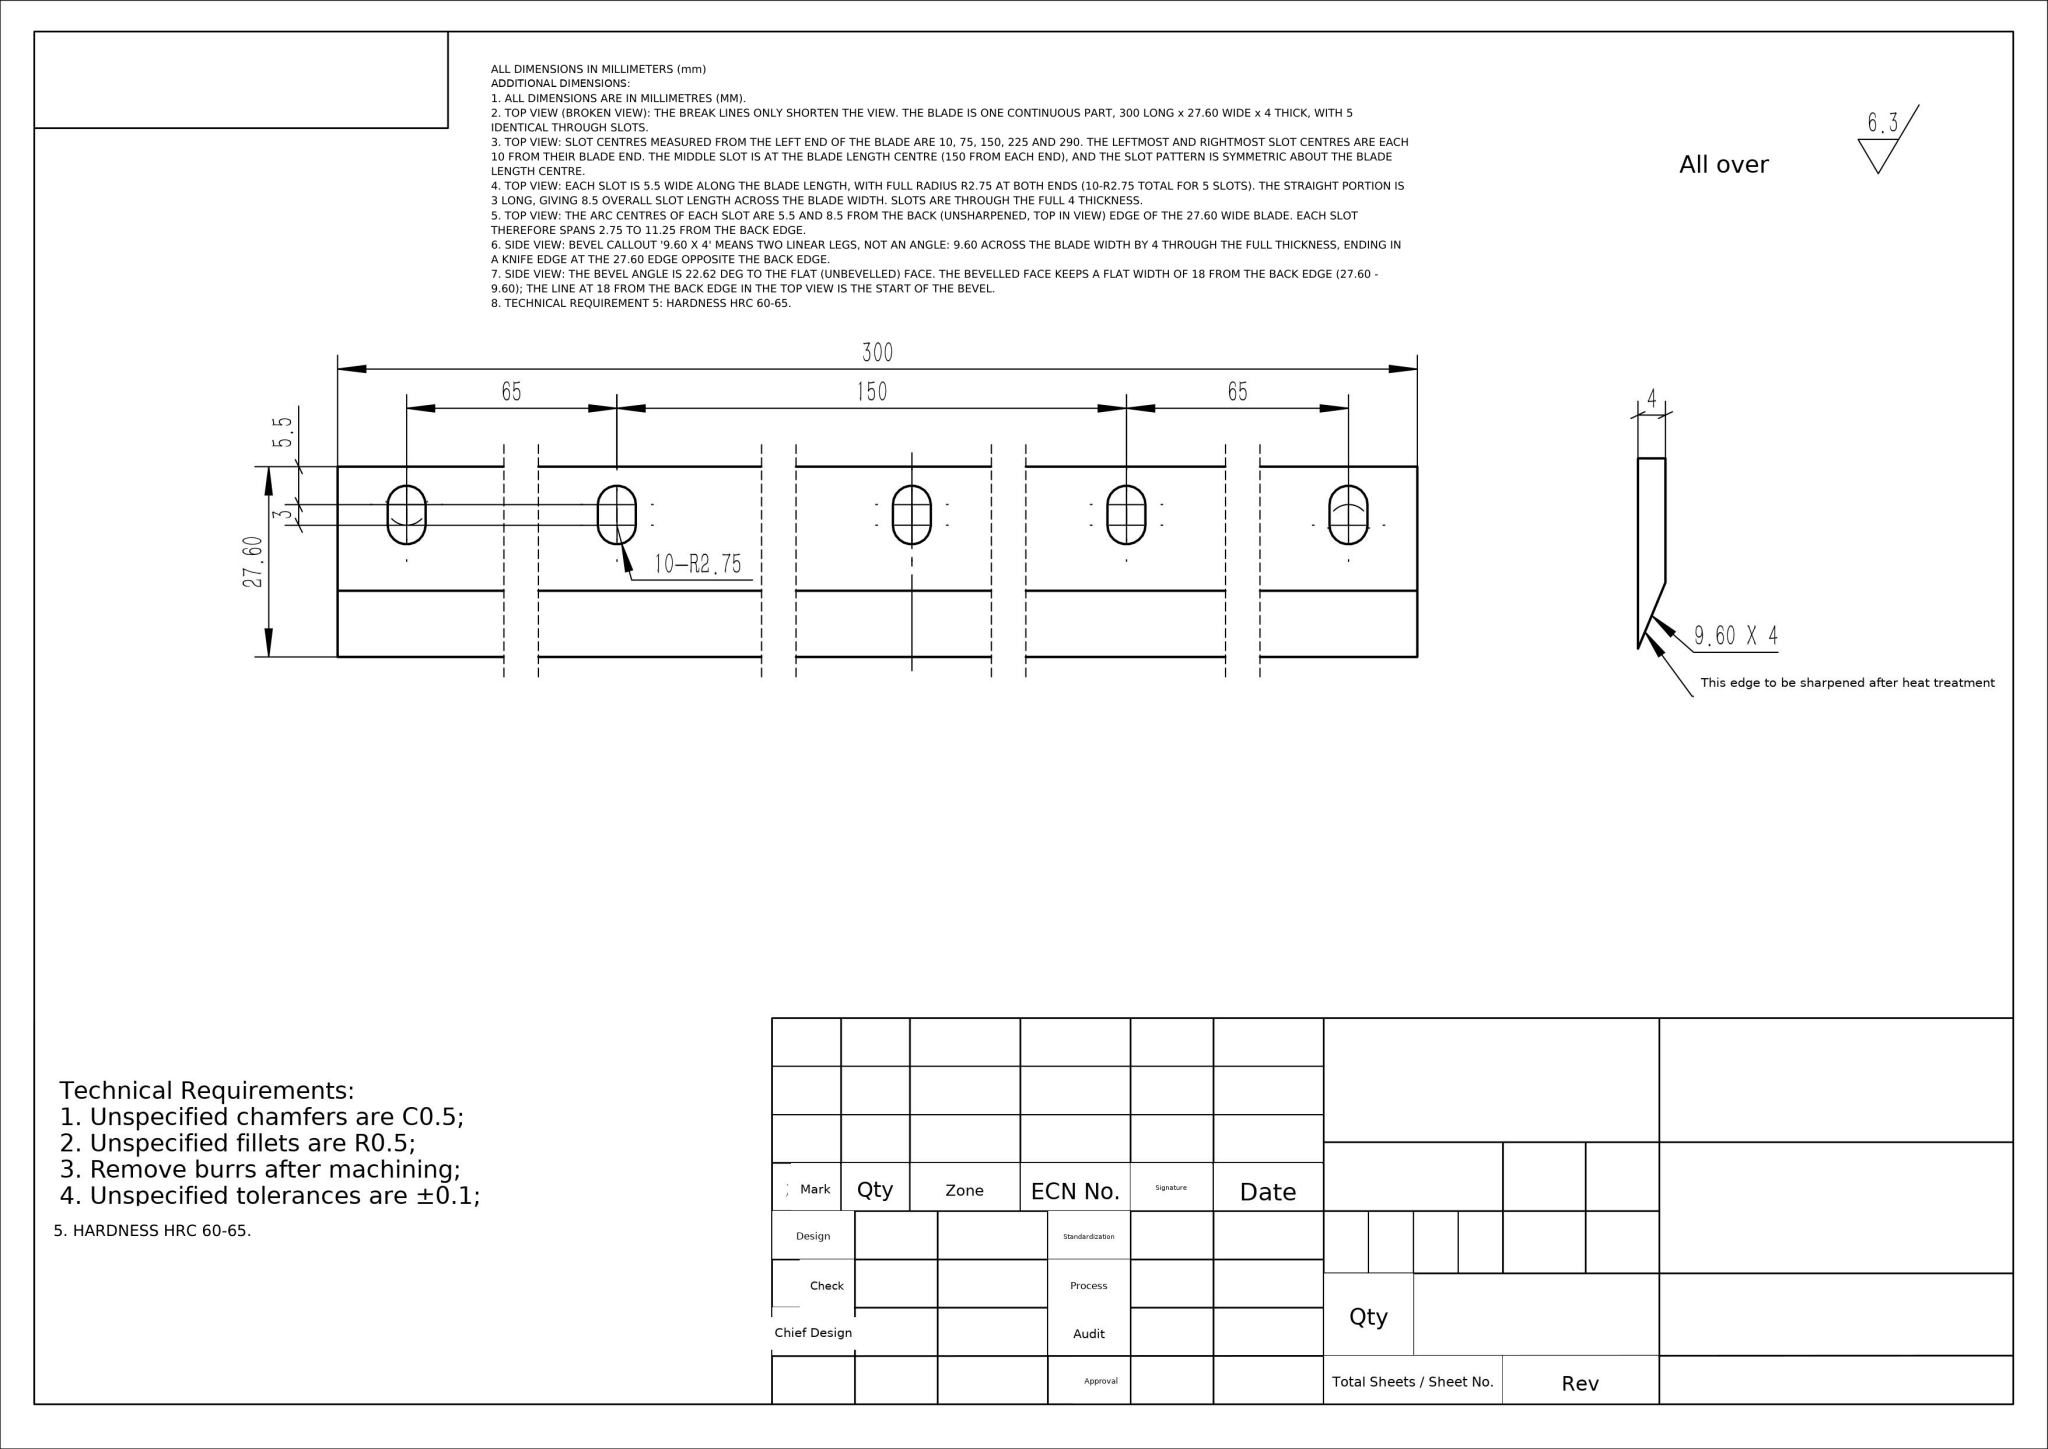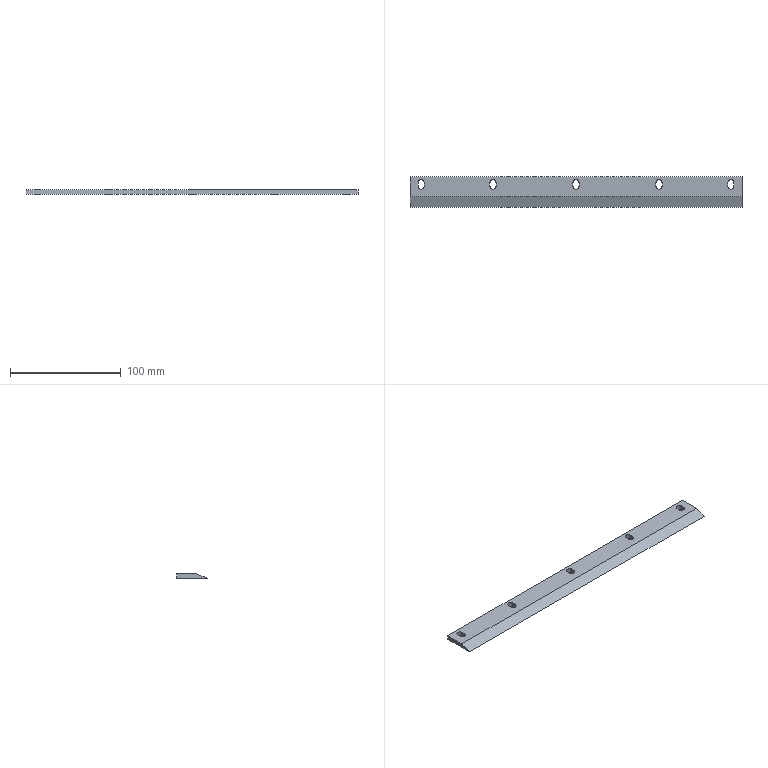Part | NX | mm | 479 | 1 solid | 26 faces | box 300 x 27.6 x 4 mm | volume 26555 mm3 | plane 16 | cylinder 10 | commonest cylinder face diameters 5.5 x10
STEP:
#1=COLOUR_RGB('',1.,1.,1.);
#2=FILL_AREA_STYLE_COLOUR('',#1);
#3=FILL_AREA_STYLE('',(#2));
#4=SURFACE_STYLE_FILL_AREA(#3);
#5=SURFACE_SIDE_STYLE('',(#4));
#6=SURFACE_STYLE_USAGE(.BOTH.,#5);
#7=PRESENTATION_STYLE_ASSIGNMENT((#6));
#8=CARTESIAN_POINT('',(-150.,0.,-2.));
#9=VERTEX_POINT('',#8);
#10=CARTESIAN_POINT('',(-150.,-27.6,-2.));
#11=VERTEX_POINT('',#10);
#12=CARTESIAN_POINT('',(-150.,0.,-2.));
#13=DIRECTION('',(0.,-1.,0.));
#14=VECTOR('',#13,1000.);
#15=LINE('',#12,#14);
#16=EDGE_CURVE('',#9,#11,#15,.T.);
#17=ORIENTED_EDGE('',*,*,#16,.T.);
#18=CARTESIAN_POINT('',(-150.,-18.,2.));
#19=VERTEX_POINT('',#18);
#20=CARTESIAN_POINT('',(-150.,-18.,2.));
#21=DIRECTION('',(0.,0.9231,0.3846));
#22=VECTOR('',#21,1000.);
#23=LINE('',#20,#22);
#24=EDGE_CURVE('',#11,#19,#23,.T.);
#25=ORIENTED_EDGE('',*,*,#24,.T.);
#26=CARTESIAN_POINT('',(-150.,0.,2.));
#27=VERTEX_POINT('',#26);
#28=CARTESIAN_POINT('',(-150.,0.,2.));
#29=DIRECTION('',(0.,-1.,0.));
#30=VECTOR('',#29,1000.);
#31=LINE('',#28,#30);
#32=EDGE_CURVE('',#27,#19,#31,.T.);
#33=ORIENTED_EDGE('',*,*,#32,.F.);
#34=CARTESIAN_POINT('',(-150.,0.,2.));
#35=DIRECTION('',(0.,0.,-1.));
#36=VECTOR('',#35,1000.);
#37=LINE('',#34,#36);
#38=EDGE_CURVE('',#27,#9,#37,.T.);
#39=ORIENTED_EDGE('',*,*,#38,.T.);
#40=EDGE_LOOP('',(#17,#25,#33,#39));
#41=FACE_OUTER_BOUND('',#40,.T.);
#42=CARTESIAN_POINT('',(-150.,0.,2.));
#43=DIRECTION('',(1.,0.,0.));
#44=DIRECTION('',(0.,0.,-1.));
#45=AXIS2_PLACEMENT_3D('',#42,#43,#44);
#46=PLANE('',#45);
#47=ADVANCED_FACE('',(#41),#46,.F.);
#48=CARTESIAN_POINT('',(150.,-18.,2.));
#49=VERTEX_POINT('',#48);
#50=CARTESIAN_POINT('',(150.,0.,2.));
#51=VERTEX_POINT('',#50);
#52=CARTESIAN_POINT('',(150.,-30.,2.));
#53=DIRECTION('',(0.,1.,0.));
#54=VECTOR('',#53,1000.);
#55=LINE('',#52,#54);
#56=EDGE_CURVE('',#49,#51,#55,.T.);
#57=ORIENTED_EDGE('',*,*,#56,.F.);
#58=CARTESIAN_POINT('',(150.,-27.6,-2.));
#59=VERTEX_POINT('',#58);
#60=CARTESIAN_POINT('',(150.,-18.,2.));
#61=DIRECTION('',(0.,-0.9231,-0.3846));
#62=VECTOR('',#61,1000.);
#63=LINE('',#60,#62);
#64=EDGE_CURVE('',#49,#59,#63,.T.);
#65=ORIENTED_EDGE('',*,*,#64,.T.);
#66=CARTESIAN_POINT('',(150.,0.,-2.));
#67=VERTEX_POINT('',#66);
#68=CARTESIAN_POINT('',(150.,-30.,-2.));
#69=DIRECTION('',(0.,1.,0.));
#70=VECTOR('',#69,1000.);
#71=LINE('',#68,#70);
#72=EDGE_CURVE('',#59,#67,#71,.T.);
#73=ORIENTED_EDGE('',*,*,#72,.T.);
#74=CARTESIAN_POINT('',(150.,0.,2.));
#75=DIRECTION('',(0.,0.,-1.));
#76=VECTOR('',#75,1000.);
#77=LINE('',#74,#76);
#78=EDGE_CURVE('',#51,#67,#77,.T.);
#79=ORIENTED_EDGE('',*,*,#78,.F.);
#80=EDGE_LOOP('',(#57,#65,#73,#79));
#81=FACE_OUTER_BOUND('',#80,.T.);
#82=CARTESIAN_POINT('',(150.,-30.,2.));
#83=DIRECTION('',(-1.,0.,0.));
#84=DIRECTION('',(0.,0.,1.));
#85=AXIS2_PLACEMENT_3D('',#82,#83,#84);
#86=PLANE('',#85);
#87=ADVANCED_FACE('',(#81),#86,.F.);
#88=CARTESIAN_POINT('',(-150.,0.,-2.));
#89=DIRECTION('',(-1.,0.,0.));
#90=VECTOR('',#89,1000.);
#91=LINE('',#88,#90);
#92=EDGE_CURVE('',#67,#9,#91,.T.);
#93=ORIENTED_EDGE('',*,*,#92,.T.);
#94=ORIENTED_EDGE('',*,*,#38,.F.);
#95=CARTESIAN_POINT('',(-150.,0.,2.));
#96=DIRECTION('',(-1.,0.,0.));
#97=VECTOR('',#96,1000.);
#98=LINE('',#95,#97);
#99=EDGE_CURVE('',#51,#27,#98,.T.);
#100=ORIENTED_EDGE('',*,*,#99,.F.);
#101=ORIENTED_EDGE('',*,*,#78,.T.);
#102=EDGE_LOOP('',(#93,#94,#100,#101));
#103=FACE_OUTER_BOUND('',#102,.T.);
#104=CARTESIAN_POINT('',(-150.,0.,2.));
#105=DIRECTION('',(0.,-1.,0.));
#106=DIRECTION('',(0.,0.,-1.));
#107=AXIS2_PLACEMENT_3D('',#104,#105,#106);
#108=PLANE('',#107);
#109=ADVANCED_FACE('',(#103),#108,.F.);
#110=CARTESIAN_POINT('',(142.75,-5.5,2.));
#111=VERTEX_POINT('',#110);
#112=CARTESIAN_POINT('',(137.25,-5.5,2.));
#113=VERTEX_POINT('',#112);
#114=CARTESIAN_POINT('',(140.,-5.5,2.));
#115=DIRECTION('',(0.,0.,1.));
#116=DIRECTION('',(-1.,0.,0.));
#117=AXIS2_PLACEMENT_3D('',#114,#115,#116);
#118=CIRCLE('',#117,2.75);
#119=EDGE_CURVE('',#111,#113,#118,.T.);
#120=ORIENTED_EDGE('',*,*,#119,.F.);
#121=CARTESIAN_POINT('',(142.75,-8.5,2.));
#122=VERTEX_POINT('',#121);
#123=CARTESIAN_POINT('',(142.75,-5.5,2.));
#124=DIRECTION('',(0.,1.,0.));
#125=VECTOR('',#124,1000.);
#126=LINE('',#123,#125);
#127=EDGE_CURVE('',#122,#111,#126,.T.);
#128=ORIENTED_EDGE('',*,*,#127,.F.);
#129=CARTESIAN_POINT('',(137.25,-8.5,2.));
#130=VERTEX_POINT('',#129);
#131=CARTESIAN_POINT('',(140.,-8.5,2.));
#132=DIRECTION('',(0.,0.,1.));
#133=DIRECTION('',(-1.,0.,0.));
#134=AXIS2_PLACEMENT_3D('',#131,#132,#133);
#135=CIRCLE('',#134,2.75);
#136=EDGE_CURVE('',#130,#122,#135,.T.);
#137=ORIENTED_EDGE('',*,*,#136,.F.);
#138=CARTESIAN_POINT('',(137.25,-5.5,2.));
#139=DIRECTION('',(0.,-1.,0.));
#140=VECTOR('',#139,1000.);
#141=LINE('',#138,#140);
#142=EDGE_CURVE('',#113,#130,#141,.T.);
#143=ORIENTED_EDGE('',*,*,#142,.F.);
#144=EDGE_LOOP('',(#120,#128,#137,#143));
#145=FACE_BOUND('',#144,.T.);
#146=CARTESIAN_POINT('',(-137.25,-5.5,2.));
#147=VERTEX_POINT('',#146);
#148=CARTESIAN_POINT('',(-142.75,-5.5,2.));
#149=VERTEX_POINT('',#148);
#150=CARTESIAN_POINT('',(-140.,-5.5,2.));
#151=DIRECTION('',(0.,0.,1.));
#152=DIRECTION('',(1.,0.,0.));
#153=AXIS2_PLACEMENT_3D('',#150,#151,#152);
#154=CIRCLE('',#153,2.75);
#155=EDGE_CURVE('',#147,#149,#154,.T.);
#156=ORIENTED_EDGE('',*,*,#155,.F.);
#157=CARTESIAN_POINT('',(-137.25,-8.5,2.));
#158=VERTEX_POINT('',#157);
#159=CARTESIAN_POINT('',(-137.25,-5.5,2.));
#160=DIRECTION('',(0.,1.,0.));
#161=VECTOR('',#160,1000.);
#162=LINE('',#159,#161);
#163=EDGE_CURVE('',#158,#147,#162,.T.);
#164=ORIENTED_EDGE('',*,*,#163,.F.);
#165=CARTESIAN_POINT('',(-142.75,-8.5,2.));
#166=VERTEX_POINT('',#165);
#167=CARTESIAN_POINT('',(-140.,-8.5,2.));
#168=DIRECTION('',(0.,0.,1.));
#169=DIRECTION('',(1.,0.,0.));
#170=AXIS2_PLACEMENT_3D('',#167,#168,#169);
#171=CIRCLE('',#170,2.75);
#172=EDGE_CURVE('',#166,#158,#171,.T.);
#173=ORIENTED_EDGE('',*,*,#172,.F.);
#174=CARTESIAN_POINT('',(-142.75,-5.5,2.));
#175=DIRECTION('',(0.,-1.,0.));
#176=VECTOR('',#175,1000.);
#177=LINE('',#174,#176);
#178=EDGE_CURVE('',#149,#166,#177,.T.);
#179=ORIENTED_EDGE('',*,*,#178,.F.);
#180=EDGE_LOOP('',(#156,#164,#173,#179));
#181=FACE_BOUND('',#180,.T.);
#182=CARTESIAN_POINT('',(2.75,-5.5,2.));
#183=VERTEX_POINT('',#182);
#184=CARTESIAN_POINT('',(-2.75,-5.5,2.));
#185=VERTEX_POINT('',#184);
#186=CARTESIAN_POINT('',(-0.,-5.5,2.));
#187=DIRECTION('',(0.,0.,1.));
#188=DIRECTION('',(1.,0.,0.));
#189=AXIS2_PLACEMENT_3D('',#186,#187,#188);
#190=CIRCLE('',#189,2.75);
#191=EDGE_CURVE('',#183,#185,#190,.T.);
#192=ORIENTED_EDGE('',*,*,#191,.F.);
#193=CARTESIAN_POINT('',(2.75,-8.5,2.));
#194=VERTEX_POINT('',#193);
#195=CARTESIAN_POINT('',(2.75,-5.5,2.));
#196=DIRECTION('',(-0.,1.,0.));
#197=VECTOR('',#196,1000.);
#198=LINE('',#195,#197);
#199=EDGE_CURVE('',#194,#183,#198,.T.);
#200=ORIENTED_EDGE('',*,*,#199,.F.);
#201=CARTESIAN_POINT('',(-2.75,-8.5,2.));
#202=VERTEX_POINT('',#201);
#203=CARTESIAN_POINT('',(0.,-8.5,2.));
#204=DIRECTION('',(0.,0.,1.));
#205=DIRECTION('',(1.,0.,0.));
#206=AXIS2_PLACEMENT_3D('',#203,#204,#205);
#207=CIRCLE('',#206,2.75);
#208=EDGE_CURVE('',#202,#194,#207,.T.);
#209=ORIENTED_EDGE('',*,*,#208,.F.);
#210=CARTESIAN_POINT('',(-2.75,-5.5,2.));
#211=DIRECTION('',(0.,-1.,0.));
#212=VECTOR('',#211,1000.);
#213=LINE('',#210,#212);
#214=EDGE_CURVE('',#185,#202,#213,.T.);
#215=ORIENTED_EDGE('',*,*,#214,.F.);
#216=EDGE_LOOP('',(#192,#200,#209,#215));
#217=FACE_BOUND('',#216,.T.);
#218=CARTESIAN_POINT('',(77.75,-5.5,2.));
#219=VERTEX_POINT('',#218);
#220=CARTESIAN_POINT('',(72.25,-5.5,2.));
#221=VERTEX_POINT('',#220);
#222=CARTESIAN_POINT('',(75.,-5.5,2.));
#223=DIRECTION('',(0.,0.,1.));
#224=DIRECTION('',(-1.,0.,0.));
#225=AXIS2_PLACEMENT_3D('',#222,#223,#224);
#226=CIRCLE('',#225,2.75);
#227=EDGE_CURVE('',#219,#221,#226,.T.);
#228=ORIENTED_EDGE('',*,*,#227,.F.);
#229=CARTESIAN_POINT('',(77.75,-8.5,2.));
#230=VERTEX_POINT('',#229);
#231=CARTESIAN_POINT('',(77.75,-5.5,2.));
#232=DIRECTION('',(0.,1.,0.));
#233=VECTOR('',#232,1000.);
#234=LINE('',#231,#233);
#235=EDGE_CURVE('',#230,#219,#234,.T.);
#236=ORIENTED_EDGE('',*,*,#235,.F.);
#237=CARTESIAN_POINT('',(72.25,-8.5,2.));
#238=VERTEX_POINT('',#237);
#239=CARTESIAN_POINT('',(75.,-8.5,2.));
#240=DIRECTION('',(0.,0.,1.));
#241=DIRECTION('',(-1.,0.,0.));
#242=AXIS2_PLACEMENT_3D('',#239,#240,#241);
#243=CIRCLE('',#242,2.75);
#244=EDGE_CURVE('',#238,#230,#243,.T.);
#245=ORIENTED_EDGE('',*,*,#244,.F.);
#246=CARTESIAN_POINT('',(72.25,-5.5,2.));
#247=DIRECTION('',(0.,-1.,0.));
#248=VECTOR('',#247,1000.);
#249=LINE('',#246,#248);
#250=EDGE_CURVE('',#221,#238,#249,.T.);
#251=ORIENTED_EDGE('',*,*,#250,.F.);
#252=EDGE_LOOP('',(#228,#236,#245,#251));
#253=FACE_BOUND('',#252,.T.);
#254=CARTESIAN_POINT('',(-72.25,-5.5,2.));
#255=VERTEX_POINT('',#254);
#256=CARTESIAN_POINT('',(-77.75,-5.5,2.));
#257=VERTEX_POINT('',#256);
#258=CARTESIAN_POINT('',(-75.,-5.5,2.));
#259=DIRECTION('',(0.,0.,1.));
#260=DIRECTION('',(1.,0.,0.));
#261=AXIS2_PLACEMENT_3D('',#258,#259,#260);
#262=CIRCLE('',#261,2.75);
#263=EDGE_CURVE('',#255,#257,#262,.T.);
#264=ORIENTED_EDGE('',*,*,#263,.F.);
#265=CARTESIAN_POINT('',(-72.25,-8.5,2.));
#266=VERTEX_POINT('',#265);
#267=CARTESIAN_POINT('',(-72.25,-5.5,2.));
#268=DIRECTION('',(0.,1.,0.));
#269=VECTOR('',#268,1000.);
#270=LINE('',#267,#269);
#271=EDGE_CURVE('',#266,#255,#270,.T.);
#272=ORIENTED_EDGE('',*,*,#271,.F.);
#273=CARTESIAN_POINT('',(-77.75,-8.5,2.));
#274=VERTEX_POINT('',#273);
#275=CARTESIAN_POINT('',(-75.,-8.5,2.));
#276=DIRECTION('',(0.,0.,1.));
#277=DIRECTION('',(1.,0.,0.));
#278=AXIS2_PLACEMENT_3D('',#275,#276,#277);
#279=CIRCLE('',#278,2.75);
#280=EDGE_CURVE('',#274,#266,#279,.T.);
#281=ORIENTED_EDGE('',*,*,#280,.F.);
#282=CARTESIAN_POINT('',(-77.75,-5.5,2.));
#283=DIRECTION('',(0.,-1.,0.));
#284=VECTOR('',#283,1000.);
#285=LINE('',#282,#284);
#286=EDGE_CURVE('',#257,#274,#285,.T.);
#287=ORIENTED_EDGE('',*,*,#286,.F.);
#288=EDGE_LOOP('',(#264,#272,#281,#287));
#289=FACE_BOUND('',#288,.T.);
#290=ORIENTED_EDGE('',*,*,#32,.T.);
#291=CARTESIAN_POINT('',(150.,-18.,2.));
#292=DIRECTION('',(1.,0.,0.));
#293=VECTOR('',#292,1000.);
#294=LINE('',#291,#293);
#295=EDGE_CURVE('',#19,#49,#294,.T.);
#296=ORIENTED_EDGE('',*,*,#295,.T.);
#297=ORIENTED_EDGE('',*,*,#56,.T.);
#298=ORIENTED_EDGE('',*,*,#99,.T.);
#299=EDGE_LOOP('',(#290,#296,#297,#298));
#300=FACE_OUTER_BOUND('',#299,.T.);
#301=CARTESIAN_POINT('',(0.,0.,2.));
#302=DIRECTION('',(0.,0.,1.));
#303=DIRECTION('',(1.,0.,0.));
#304=AXIS2_PLACEMENT_3D('',#301,#302,#303);
#305=PLANE('',#304);
#306=ADVANCED_FACE('',(#145,#181,#217,#253,#289,#300),#305,.T.);
#307=CARTESIAN_POINT('',(142.75,-8.5,-2.));
#308=VERTEX_POINT('',#307);
#309=CARTESIAN_POINT('',(142.75,-5.5,-2.));
#310=VERTEX_POINT('',#309);
#311=CARTESIAN_POINT('',(142.75,-5.5,-2.));
#312=DIRECTION('',(0.,1.,0.));
#313=VECTOR('',#312,1000.);
#314=LINE('',#311,#313);
#315=EDGE_CURVE('',#308,#310,#314,.T.);
#316=ORIENTED_EDGE('',*,*,#315,.T.);
#317=CARTESIAN_POINT('',(137.25,-5.5,-2.));
#318=VERTEX_POINT('',#317);
#319=CARTESIAN_POINT('',(140.,-5.5,-2.));
#320=DIRECTION('',(0.,0.,1.));
#321=DIRECTION('',(-1.,0.,0.));
#322=AXIS2_PLACEMENT_3D('',#319,#320,#321);
#323=CIRCLE('',#322,2.75);
#324=EDGE_CURVE('',#310,#318,#323,.T.);
#325=ORIENTED_EDGE('',*,*,#324,.T.);
#326=CARTESIAN_POINT('',(137.25,-8.5,-2.));
#327=VERTEX_POINT('',#326);
#328=CARTESIAN_POINT('',(137.25,-5.5,-2.));
#329=DIRECTION('',(0.,-1.,0.));
#330=VECTOR('',#329,1000.);
#331=LINE('',#328,#330);
#332=EDGE_CURVE('',#318,#327,#331,.T.);
#333=ORIENTED_EDGE('',*,*,#332,.T.);
#334=CARTESIAN_POINT('',(140.,-8.5,-2.));
#335=DIRECTION('',(0.,0.,1.));
#336=DIRECTION('',(-1.,0.,0.));
#337=AXIS2_PLACEMENT_3D('',#334,#335,#336);
#338=CIRCLE('',#337,2.75);
#339=EDGE_CURVE('',#327,#308,#338,.T.);
#340=ORIENTED_EDGE('',*,*,#339,.T.);
#341=EDGE_LOOP('',(#316,#325,#333,#340));
#342=FACE_BOUND('',#341,.T.);
#343=CARTESIAN_POINT('',(-137.25,-8.5,-2.));
#344=VERTEX_POINT('',#343);
#345=CARTESIAN_POINT('',(-137.25,-5.5,-2.));
#346=VERTEX_POINT('',#345);
#347=CARTESIAN_POINT('',(-137.25,-5.5,-2.));
#348=DIRECTION('',(0.,1.,0.));
#349=VECTOR('',#348,1000.);
#350=LINE('',#347,#349);
#351=EDGE_CURVE('',#344,#346,#350,.T.);
#352=ORIENTED_EDGE('',*,*,#351,.T.);
#353=CARTESIAN_POINT('',(-142.75,-5.5,-2.));
#354=VERTEX_POINT('',#353);
#355=CARTESIAN_POINT('',(-140.,-5.5,-2.));
#356=DIRECTION('',(0.,0.,1.));
#357=DIRECTION('',(1.,0.,0.));
#358=AXIS2_PLACEMENT_3D('',#355,#356,#357);
#359=CIRCLE('',#358,2.75);
#360=EDGE_CURVE('',#346,#354,#359,.T.);
#361=ORIENTED_EDGE('',*,*,#360,.T.);
#362=CARTESIAN_POINT('',(-142.75,-8.5,-2.));
#363=VERTEX_POINT('',#362);
#364=CARTESIAN_POINT('',(-142.75,-5.5,-2.));
#365=DIRECTION('',(0.,-1.,0.));
#366=VECTOR('',#365,1000.);
#367=LINE('',#364,#366);
#368=EDGE_CURVE('',#354,#363,#367,.T.);
#369=ORIENTED_EDGE('',*,*,#368,.T.);
#370=CARTESIAN_POINT('',(-140.,-8.5,-2.));
#371=DIRECTION('',(0.,0.,1.));
#372=DIRECTION('',(1.,0.,0.));
#373=AXIS2_PLACEMENT_3D('',#370,#371,#372);
#374=CIRCLE('',#373,2.75);
#375=EDGE_CURVE('',#363,#344,#374,.T.);
#376=ORIENTED_EDGE('',*,*,#375,.T.);
#377=EDGE_LOOP('',(#352,#361,#369,#376));
#378=FACE_BOUND('',#377,.T.);
#379=CARTESIAN_POINT('',(2.75,-8.5,-2.));
#380=VERTEX_POINT('',#379);
#381=CARTESIAN_POINT('',(2.75,-5.5,-2.));
#382=VERTEX_POINT('',#381);
#383=CARTESIAN_POINT('',(2.75,-5.5,-2.));
#384=DIRECTION('',(-0.,1.,0.));
#385=VECTOR('',#384,1000.);
#386=LINE('',#383,#385);
#387=EDGE_CURVE('',#380,#382,#386,.T.);
#388=ORIENTED_EDGE('',*,*,#387,.T.);
#389=CARTESIAN_POINT('',(-2.75,-5.5,-2.));
#390=VERTEX_POINT('',#389);
#391=CARTESIAN_POINT('',(-0.,-5.5,-2.));
#392=DIRECTION('',(0.,0.,1.));
#393=DIRECTION('',(1.,0.,0.));
#394=AXIS2_PLACEMENT_3D('',#391,#392,#393);
#395=CIRCLE('',#394,2.75);
#396=EDGE_CURVE('',#382,#390,#395,.T.);
#397=ORIENTED_EDGE('',*,*,#396,.T.);
#398=CARTESIAN_POINT('',(-2.75,-8.5,-2.));
#399=VERTEX_POINT('',#398);
#400=CARTESIAN_POINT('',(-2.75,-5.5,-2.));
#401=DIRECTION('',(0.,-1.,0.));
#402=VECTOR('',#401,1000.);
#403=LINE('',#400,#402);
#404=EDGE_CURVE('',#390,#399,#403,.T.);
#405=ORIENTED_EDGE('',*,*,#404,.T.);
#406=CARTESIAN_POINT('',(0.,-8.5,-2.));
#407=DIRECTION('',(0.,0.,1.));
#408=DIRECTION('',(1.,0.,0.));
#409=AXIS2_PLACEMENT_3D('',#406,#407,#408);
#410=CIRCLE('',#409,2.75);
#411=EDGE_CURVE('',#399,#380,#410,.T.);
#412=ORIENTED_EDGE('',*,*,#411,.T.);
#413=EDGE_LOOP('',(#388,#397,#405,#412));
#414=FACE_BOUND('',#413,.T.);
#415=CARTESIAN_POINT('',(77.75,-8.5,-2.));
#416=VERTEX_POINT('',#415);
#417=CARTESIAN_POINT('',(77.75,-5.5,-2.));
#418=VERTEX_POINT('',#417);
#419=CARTESIAN_POINT('',(77.75,-5.5,-2.));
#420=DIRECTION('',(0.,1.,0.));
#421=VECTOR('',#420,1000.);
#422=LINE('',#419,#421);
#423=EDGE_CURVE('',#416,#418,#422,.T.);
#424=ORIENTED_EDGE('',*,*,#423,.T.);
#425=CARTESIAN_POINT('',(72.25,-5.5,-2.));
#426=VERTEX_POINT('',#425);
#427=CARTESIAN_POINT('',(75.,-5.5,-2.));
#428=DIRECTION('',(0.,0.,1.));
#429=DIRECTION('',(-1.,0.,0.));
#430=AXIS2_PLACEMENT_3D('',#427,#428,#429);
#431=CIRCLE('',#430,2.75);
#432=EDGE_CURVE('',#418,#426,#431,.T.);
#433=ORIENTED_EDGE('',*,*,#432,.T.);
#434=CARTESIAN_POINT('',(72.25,-8.5,-2.));
#435=VERTEX_POINT('',#434);
#436=CARTESIAN_POINT('',(72.25,-5.5,-2.));
#437=DIRECTION('',(0.,-1.,0.));
#438=VECTOR('',#437,1000.);
#439=LINE('',#436,#438);
#440=EDGE_CURVE('',#426,#435,#439,.T.);
#441=ORIENTED_EDGE('',*,*,#440,.T.);
#442=CARTESIAN_POINT('',(75.,-8.5,-2.));
#443=DIRECTION('',(0.,0.,1.));
#444=DIRECTION('',(-1.,0.,0.));
#445=AXIS2_PLACEMENT_3D('',#442,#443,#444);
#446=CIRCLE('',#445,2.75);
#447=EDGE_CURVE('',#435,#416,#446,.T.);
#448=ORIENTED_EDGE('',*,*,#447,.T.);
#449=EDGE_LOOP('',(#424,#433,#441,#448));
#450=FACE_BOUND('',#449,.T.);
#451=CARTESIAN_POINT('',(-72.25,-8.5,-2.));
#452=VERTEX_POINT('',#451);
#453=CARTESIAN_POINT('',(-72.25,-5.5,-2.));
#454=VERTEX_POINT('',#453);
#455=CARTESIAN_POINT('',(-72.25,-5.5,-2.));
#456=DIRECTION('',(0.,1.,0.));
#457=VECTOR('',#456,1000.);
#458=LINE('',#455,#457);
#459=EDGE_CURVE('',#452,#454,#458,.T.);
#460=ORIENTED_EDGE('',*,*,#459,.T.);
#461=CARTESIAN_POINT('',(-77.75,-5.5,-2.));
#462=VERTEX_POINT('',#461);
#463=CARTESIAN_POINT('',(-75.,-5.5,-2.));
#464=DIRECTION('',(0.,0.,1.));
#465=DIRECTION('',(1.,0.,0.));
#466=AXIS2_PLACEMENT_3D('',#463,#464,#465);
#467=CIRCLE('',#466,2.75);
#468=EDGE_CURVE('',#454,#462,#467,.T.);
#469=ORIENTED_EDGE('',*,*,#468,.T.);
#470=CARTESIAN_POINT('',(-77.75,-8.5,-2.));
#471=VERTEX_POINT('',#470);
#472=CARTESIAN_POINT('',(-77.75,-5.5,-2.));
#473=DIRECTION('',(0.,-1.,0.));
#474=VECTOR('',#473,1000.);
#475=LINE('',#472,#474);
#476=EDGE_CURVE('',#462,#471,#475,.T.);
#477=ORIENTED_EDGE('',*,*,#476,.T.);
#478=CARTESIAN_POINT('',(-75.,-8.5,-2.));
#479=DIRECTION('',(0.,0.,1.));
#480=DIRECTION('',(1.,0.,0.));
#481=AXIS2_PLACEMENT_3D('',#478,#479,#480);
#482=CIRCLE('',#481,2.75);
#483=EDGE_CURVE('',#471,#452,#482,.T.);
#484=ORIENTED_EDGE('',*,*,#483,.T.);
#485=EDGE_LOOP('',(#460,#469,#477,#484));
#486=FACE_BOUND('',#485,.T.);
#487=ORIENTED_EDGE('',*,*,#72,.F.);
#488=CARTESIAN_POINT('',(0.,-27.6,-2.));
#489=DIRECTION('',(-1.,0.,0.));
#490=VECTOR('',#489,1000.);
#491=LINE('',#488,#490);
#492=EDGE_CURVE('',#59,#11,#491,.T.);
#493=ORIENTED_EDGE('',*,*,#492,.T.);
#494=ORIENTED_EDGE('',*,*,#16,.F.);
#495=ORIENTED_EDGE('',*,*,#92,.F.);
#496=EDGE_LOOP('',(#487,#493,#494,#495));
#497=FACE_OUTER_BOUND('',#496,.T.);
#498=CARTESIAN_POINT('',(0.,0.,-2.));
#499=DIRECTION('',(0.,0.,1.));
#500=DIRECTION('',(1.,0.,0.));
#501=AXIS2_PLACEMENT_3D('',#498,#499,#500);
#502=PLANE('',#501);
#503=ADVANCED_FACE('',(#342,#378,#414,#450,#486,#497),#502,.F.);
#504=ORIENTED_EDGE('',*,*,#24,.F.);
#505=ORIENTED_EDGE('',*,*,#492,.F.);
#506=ORIENTED_EDGE('',*,*,#64,.F.);
#507=ORIENTED_EDGE('',*,*,#295,.F.);
#508=EDGE_LOOP('',(#504,#505,#506,#507));
#509=FACE_OUTER_BOUND('',#508,.T.);
#510=CARTESIAN_POINT('',(0.,-18.,2.));
#511=DIRECTION('',(0.,-0.3846,0.9231));
#512=DIRECTION('',(-1.,0.,0.));
#513=AXIS2_PLACEMENT_3D('',#510,#511,#512);
#514=PLANE('',#513);
#515=ADVANCED_FACE('',(#509),#514,.T.);
#516=ORIENTED_EDGE('',*,*,#263,.T.);
#517=CARTESIAN_POINT('',(-77.75,-5.5,-2.));
#518=DIRECTION('',(0.,0.,1.));
#519=VECTOR('',#518,1000.);
#520=LINE('',#517,#519);
#521=EDGE_CURVE('',#462,#257,#520,.T.);
#522=ORIENTED_EDGE('',*,*,#521,.F.);
#523=ORIENTED_EDGE('',*,*,#468,.F.);
#524=CARTESIAN_POINT('',(-72.25,-5.5,-2.));
#525=DIRECTION('',(0.,0.,1.));
#526=VECTOR('',#525,1000.);
#527=LINE('',#524,#526);
#528=EDGE_CURVE('',#454,#255,#527,.T.);
#529=ORIENTED_EDGE('',*,*,#528,.T.);
#530=EDGE_LOOP('',(#516,#522,#523,#529));
#531=FACE_OUTER_BOUND('',#530,.T.);
#532=CARTESIAN_POINT('',(-75.,-5.5,-2.));
#533=DIRECTION('',(0.,0.,1.));
#534=DIRECTION('',(1.,0.,0.));
#535=AXIS2_PLACEMENT_3D('',#532,#533,#534);
#536=CYLINDRICAL_SURFACE('',#535,2.75);
#537=ADVANCED_FACE('',(#531),#536,.F.);
#538=ORIENTED_EDGE('',*,*,#271,.T.);
#539=ORIENTED_EDGE('',*,*,#528,.F.);
#540=ORIENTED_EDGE('',*,*,#459,.F.);
#541=CARTESIAN_POINT('',(-72.25,-8.5,-2.));
#542=DIRECTION('',(0.,0.,1.));
#543=VECTOR('',#542,1000.);
#544=LINE('',#541,#543);
#545=EDGE_CURVE('',#452,#266,#544,.T.);
#546=ORIENTED_EDGE('',*,*,#545,.T.);
#547=EDGE_LOOP('',(#538,#539,#540,#546));
#548=FACE_OUTER_BOUND('',#547,.T.);
#549=CARTESIAN_POINT('',(-72.25,-5.5,-2.));
#550=DIRECTION('',(1.,0.,0.));
#551=DIRECTION('',(0.,0.,-1.));
#552=AXIS2_PLACEMENT_3D('',#549,#550,#551);
#553=PLANE('',#552);
#554=ADVANCED_FACE('',(#548),#553,.F.);
#555=ORIENTED_EDGE('',*,*,#280,.T.);
#556=ORIENTED_EDGE('',*,*,#545,.F.);
#557=ORIENTED_EDGE('',*,*,#483,.F.);
#558=CARTESIAN_POINT('',(-77.75,-8.5,-2.));
#559=DIRECTION('',(0.,0.,1.));
#560=VECTOR('',#559,1000.);
#561=LINE('',#558,#560);
#562=EDGE_CURVE('',#471,#274,#561,.T.);
#563=ORIENTED_EDGE('',*,*,#562,.T.);
#564=EDGE_LOOP('',(#555,#556,#557,#563));
#565=FACE_OUTER_BOUND('',#564,.T.);
#566=CARTESIAN_POINT('',(-75.,-8.5,-2.));
#567=DIRECTION('',(0.,0.,1.));
#568=DIRECTION('',(1.,0.,0.));
#569=AXIS2_PLACEMENT_3D('',#566,#567,#568);
#570=CYLINDRICAL_SURFACE('',#569,2.75);
#571=ADVANCED_FACE('',(#565),#570,.F.);
#572=ORIENTED_EDGE('',*,*,#286,.T.);
#573=ORIENTED_EDGE('',*,*,#562,.F.);
#574=ORIENTED_EDGE('',*,*,#476,.F.);
#575=ORIENTED_EDGE('',*,*,#521,.T.);
#576=EDGE_LOOP('',(#572,#573,#574,#575));
#577=FACE_OUTER_BOUND('',#576,.T.);
#578=CARTESIAN_POINT('',(-77.75,-5.5,-2.));
#579=DIRECTION('',(-1.,0.,0.));
#580=DIRECTION('',(0.,0.,1.));
#581=AXIS2_PLACEMENT_3D('',#578,#579,#580);
#582=PLANE('',#581);
#583=ADVANCED_FACE('',(#577),#582,.F.);
#584=ORIENTED_EDGE('',*,*,#227,.T.);
#585=CARTESIAN_POINT('',(72.25,-5.5,-2.));
#586=DIRECTION('',(0.,0.,1.));
#587=VECTOR('',#586,1000.);
#588=LINE('',#585,#587);
#589=EDGE_CURVE('',#426,#221,#588,.T.);
#590=ORIENTED_EDGE('',*,*,#589,.F.);
#591=ORIENTED_EDGE('',*,*,#432,.F.);
#592=CARTESIAN_POINT('',(77.75,-5.5,-2.));
#593=DIRECTION('',(0.,0.,1.));
#594=VECTOR('',#593,1000.);
#595=LINE('',#592,#594);
#596=EDGE_CURVE('',#418,#219,#595,.T.);
#597=ORIENTED_EDGE('',*,*,#596,.T.);
#598=EDGE_LOOP('',(#584,#590,#591,#597));
#599=FACE_OUTER_BOUND('',#598,.T.);
#600=CARTESIAN_POINT('',(75.,-5.5,-2.));
#601=DIRECTION('',(0.,0.,1.));
#602=DIRECTION('',(1.,0.,0.));
#603=AXIS2_PLACEMENT_3D('',#600,#601,#602);
#604=CYLINDRICAL_SURFACE('',#603,2.75);
#605=ADVANCED_FACE('',(#599),#604,.F.);
#606=ORIENTED_EDGE('',*,*,#235,.T.);
#607=ORIENTED_EDGE('',*,*,#596,.F.);
#608=ORIENTED_EDGE('',*,*,#423,.F.);
#609=CARTESIAN_POINT('',(77.75,-8.5,-2.));
#610=DIRECTION('',(0.,0.,1.));
#611=VECTOR('',#610,1000.);
#612=LINE('',#609,#611);
#613=EDGE_CURVE('',#416,#230,#612,.T.);
#614=ORIENTED_EDGE('',*,*,#613,.T.);
#615=EDGE_LOOP('',(#606,#607,#608,#614));
#616=FACE_OUTER_BOUND('',#615,.T.);
#617=CARTESIAN_POINT('',(77.75,-5.5,-2.));
#618=DIRECTION('',(1.,0.,0.));
#619=DIRECTION('',(0.,0.,-1.));
#620=AXIS2_PLACEMENT_3D('',#617,#618,#619);
#621=PLANE('',#620);
#622=ADVANCED_FACE('',(#616),#621,.F.);
#623=ORIENTED_EDGE('',*,*,#244,.T.);
#624=ORIENTED_EDGE('',*,*,#613,.F.);
#625=ORIENTED_EDGE('',*,*,#447,.F.);
#626=CARTESIAN_POINT('',(72.25,-8.5,-2.));
#627=DIRECTION('',(0.,0.,1.));
#628=VECTOR('',#627,1000.);
#629=LINE('',#626,#628);
#630=EDGE_CURVE('',#435,#238,#629,.T.);
#631=ORIENTED_EDGE('',*,*,#630,.T.);
#632=EDGE_LOOP('',(#623,#624,#625,#631));
#633=FACE_OUTER_BOUND('',#632,.T.);
#634=CARTESIAN_POINT('',(75.,-8.5,-2.));
#635=DIRECTION('',(0.,0.,1.));
#636=DIRECTION('',(1.,0.,0.));
#637=AXIS2_PLACEMENT_3D('',#634,#635,#636);
#638=CYLINDRICAL_SURFACE('',#637,2.75);
#639=ADVANCED_FACE('',(#633),#638,.F.);
#640=ORIENTED_EDGE('',*,*,#250,.T.);
#641=ORIENTED_EDGE('',*,*,#630,.F.);
#642=ORIENTED_EDGE('',*,*,#440,.F.);
#643=ORIENTED_EDGE('',*,*,#589,.T.);
#644=EDGE_LOOP('',(#640,#641,#642,#643));
#645=FACE_OUTER_BOUND('',#644,.T.);
#646=CARTESIAN_POINT('',(72.25,-5.5,-2.));
#647=DIRECTION('',(-1.,0.,0.));
#648=DIRECTION('',(0.,0.,1.));
#649=AXIS2_PLACEMENT_3D('',#646,#647,#648);
#650=PLANE('',#649);
#651=ADVANCED_FACE('',(#645),#650,.F.);
#652=ORIENTED_EDGE('',*,*,#191,.T.);
#653=CARTESIAN_POINT('',(-2.75,-5.5,-2.));
#654=DIRECTION('',(0.,0.,1.));
#655=VECTOR('',#654,1000.);
#656=LINE('',#653,#655);
#657=EDGE_CURVE('',#390,#185,#656,.T.);
#658=ORIENTED_EDGE('',*,*,#657,.F.);
#659=ORIENTED_EDGE('',*,*,#396,.F.);
#660=CARTESIAN_POINT('',(2.75,-5.5,-2.));
#661=DIRECTION('',(0.,0.,1.));
#662=VECTOR('',#661,1000.);
#663=LINE('',#660,#662);
#664=EDGE_CURVE('',#382,#183,#663,.T.);
#665=ORIENTED_EDGE('',*,*,#664,.T.);
#666=EDGE_LOOP('',(#652,#658,#659,#665));
#667=FACE_OUTER_BOUND('',#666,.T.);
#668=CARTESIAN_POINT('',(-0.,-5.5,-2.));
#669=DIRECTION('',(0.,0.,1.));
#670=DIRECTION('',(1.,0.,0.));
#671=AXIS2_PLACEMENT_3D('',#668,#669,#670);
#672=CYLINDRICAL_SURFACE('',#671,2.75);
#673=ADVANCED_FACE('',(#667),#672,.F.);
#674=ORIENTED_EDGE('',*,*,#199,.T.);
#675=ORIENTED_EDGE('',*,*,#664,.F.);
#676=ORIENTED_EDGE('',*,*,#387,.F.);
#677=CARTESIAN_POINT('',(2.75,-8.5,-2.));
#678=DIRECTION('',(0.,0.,1.));
#679=VECTOR('',#678,1000.);
#680=LINE('',#677,#679);
#681=EDGE_CURVE('',#380,#194,#680,.T.);
#682=ORIENTED_EDGE('',*,*,#681,.T.);
#683=EDGE_LOOP('',(#674,#675,#676,#682));
#684=FACE_OUTER_BOUND('',#683,.T.);
#685=CARTESIAN_POINT('',(2.75,-5.5,-2.));
#686=DIRECTION('',(1.,0.,0.));
#687=DIRECTION('',(-0.,1.,0.));
#688=AXIS2_PLACEMENT_3D('',#685,#686,#687);
#689=PLANE('',#688);
#690=ADVANCED_FACE('',(#684),#689,.F.);
#691=ORIENTED_EDGE('',*,*,#208,.T.);
#692=ORIENTED_EDGE('',*,*,#681,.F.);
#693=ORIENTED_EDGE('',*,*,#411,.F.);
#694=CARTESIAN_POINT('',(-2.75,-8.5,-2.));
#695=DIRECTION('',(0.,0.,1.));
#696=VECTOR('',#695,1000.);
#697=LINE('',#694,#696);
#698=EDGE_CURVE('',#399,#202,#697,.T.);
#699=ORIENTED_EDGE('',*,*,#698,.T.);
#700=EDGE_LOOP('',(#691,#692,#693,#699));
#701=FACE_OUTER_BOUND('',#700,.T.);
#702=CARTESIAN_POINT('',(0.,-8.5,-2.));
#703=DIRECTION('',(0.,0.,1.));
#704=DIRECTION('',(1.,0.,0.));
#705=AXIS2_PLACEMENT_3D('',#702,#703,#704);
#706=CYLINDRICAL_SURFACE('',#705,2.75);
#707=ADVANCED_FACE('',(#701),#706,.F.);
#708=ORIENTED_EDGE('',*,*,#214,.T.);
#709=ORIENTED_EDGE('',*,*,#698,.F.);
#710=ORIENTED_EDGE('',*,*,#404,.F.);
#711=ORIENTED_EDGE('',*,*,#657,.T.);
#712=EDGE_LOOP('',(#708,#709,#710,#711));
#713=FACE_OUTER_BOUND('',#712,.T.);
#714=CARTESIAN_POINT('',(-2.75,-5.5,-2.));
#715=DIRECTION('',(-1.,-0.,0.));
#716=DIRECTION('',(0.,-1.,0.));
#717=AXIS2_PLACEMENT_3D('',#714,#715,#716);
#718=PLANE('',#717);
#719=ADVANCED_FACE('',(#713),#718,.F.);
#720=ORIENTED_EDGE('',*,*,#155,.T.);
#721=CARTESIAN_POINT('',(-142.75,-5.5,-2.));
#722=DIRECTION('',(0.,0.,1.));
#723=VECTOR('',#722,1000.);
#724=LINE('',#721,#723);
#725=EDGE_CURVE('',#354,#149,#724,.T.);
#726=ORIENTED_EDGE('',*,*,#725,.F.);
#727=ORIENTED_EDGE('',*,*,#360,.F.);
#728=CARTESIAN_POINT('',(-137.25,-5.5,-2.));
#729=DIRECTION('',(0.,0.,1.));
#730=VECTOR('',#729,1000.);
#731=LINE('',#728,#730);
#732=EDGE_CURVE('',#346,#147,#731,.T.);
#733=ORIENTED_EDGE('',*,*,#732,.T.);
#734=EDGE_LOOP('',(#720,#726,#727,#733));
#735=FACE_OUTER_BOUND('',#734,.T.);
#736=CARTESIAN_POINT('',(-140.,-5.5,-2.));
#737=DIRECTION('',(0.,0.,1.));
#738=DIRECTION('',(1.,0.,0.));
#739=AXIS2_PLACEMENT_3D('',#736,#737,#738);
#740=CYLINDRICAL_SURFACE('',#739,2.75);
#741=ADVANCED_FACE('',(#735),#740,.F.);
#742=ORIENTED_EDGE('',*,*,#163,.T.);
#743=ORIENTED_EDGE('',*,*,#732,.F.);
#744=ORIENTED_EDGE('',*,*,#351,.F.);
#745=CARTESIAN_POINT('',(-137.25,-8.5,-2.));
#746=DIRECTION('',(0.,0.,1.));
#747=VECTOR('',#746,1000.);
#748=LINE('',#745,#747);
#749=EDGE_CURVE('',#344,#158,#748,.T.);
#750=ORIENTED_EDGE('',*,*,#749,.T.);
#751=EDGE_LOOP('',(#742,#743,#744,#750));
#752=FACE_OUTER_BOUND('',#751,.T.);
#753=CARTESIAN_POINT('',(-137.25,-5.5,-2.));
#754=DIRECTION('',(1.,0.,0.));
#755=DIRECTION('',(0.,0.,-1.));
#756=AXIS2_PLACEMENT_3D('',#753,#754,#755);
#757=PLANE('',#756);
#758=ADVANCED_FACE('',(#752),#757,.F.);
#759=ORIENTED_EDGE('',*,*,#172,.T.);
#760=ORIENTED_EDGE('',*,*,#749,.F.);
#761=ORIENTED_EDGE('',*,*,#375,.F.);
#762=CARTESIAN_POINT('',(-142.75,-8.5,-2.));
#763=DIRECTION('',(0.,0.,1.));
#764=VECTOR('',#763,1000.);
#765=LINE('',#762,#764);
#766=EDGE_CURVE('',#363,#166,#765,.T.);
#767=ORIENTED_EDGE('',*,*,#766,.T.);
#768=EDGE_LOOP('',(#759,#760,#761,#767));
#769=FACE_OUTER_BOUND('',#768,.T.);
#770=CARTESIAN_POINT('',(-140.,-8.5,-2.));
#771=DIRECTION('',(0.,0.,1.));
#772=DIRECTION('',(1.,0.,0.));
#773=AXIS2_PLACEMENT_3D('',#770,#771,#772);
#774=CYLINDRICAL_SURFACE('',#773,2.75);
#775=ADVANCED_FACE('',(#769),#774,.F.);
#776=ORIENTED_EDGE('',*,*,#178,.T.);
#777=ORIENTED_EDGE('',*,*,#766,.F.);
#778=ORIENTED_EDGE('',*,*,#368,.F.);
#779=ORIENTED_EDGE('',*,*,#725,.T.);
#780=EDGE_LOOP('',(#776,#777,#778,#779));
#781=FACE_OUTER_BOUND('',#780,.T.);
#782=CARTESIAN_POINT('',(-142.75,-5.5,-2.));
#783=DIRECTION('',(-1.,0.,0.));
#784=DIRECTION('',(0.,0.,1.));
#785=AXIS2_PLACEMENT_3D('',#782,#783,#784);
#786=PLANE('',#785);
#787=ADVANCED_FACE('',(#781),#786,.F.);
#788=ORIENTED_EDGE('',*,*,#119,.T.);
#789=CARTESIAN_POINT('',(137.25,-5.5,-2.));
#790=DIRECTION('',(0.,0.,1.));
#791=VECTOR('',#790,1000.);
#792=LINE('',#789,#791);
#793=EDGE_CURVE('',#318,#113,#792,.T.);
#794=ORIENTED_EDGE('',*,*,#793,.F.);
#795=ORIENTED_EDGE('',*,*,#324,.F.);
#796=CARTESIAN_POINT('',(142.75,-5.5,-2.));
#797=DIRECTION('',(0.,0.,1.));
#798=VECTOR('',#797,1000.);
#799=LINE('',#796,#798);
#800=EDGE_CURVE('',#310,#111,#799,.T.);
#801=ORIENTED_EDGE('',*,*,#800,.T.);
#802=EDGE_LOOP('',(#788,#794,#795,#801));
#803=FACE_OUTER_BOUND('',#802,.T.);
#804=CARTESIAN_POINT('',(140.,-5.5,-2.));
#805=DIRECTION('',(0.,0.,1.));
#806=DIRECTION('',(1.,0.,0.));
#807=AXIS2_PLACEMENT_3D('',#804,#805,#806);
#808=CYLINDRICAL_SURFACE('',#807,2.75);
#809=ADVANCED_FACE('',(#803),#808,.F.);
#810=ORIENTED_EDGE('',*,*,#127,.T.);
#811=ORIENTED_EDGE('',*,*,#800,.F.);
#812=ORIENTED_EDGE('',*,*,#315,.F.);
#813=CARTESIAN_POINT('',(142.75,-8.5,-2.));
#814=DIRECTION('',(0.,0.,1.));
#815=VECTOR('',#814,1000.);
#816=LINE('',#813,#815);
#817=EDGE_CURVE('',#308,#122,#816,.T.);
#818=ORIENTED_EDGE('',*,*,#817,.T.);
#819=EDGE_LOOP('',(#810,#811,#812,#818));
#820=FACE_OUTER_BOUND('',#819,.T.);
#821=CARTESIAN_POINT('',(142.75,-5.5,-2.));
#822=DIRECTION('',(1.,0.,0.));
#823=DIRECTION('',(0.,0.,-1.));
#824=AXIS2_PLACEMENT_3D('',#821,#822,#823);
#825=PLANE('',#824);
#826=ADVANCED_FACE('',(#820),#825,.F.);
#827=ORIENTED_EDGE('',*,*,#136,.T.);
#828=ORIENTED_EDGE('',*,*,#817,.F.);
#829=ORIENTED_EDGE('',*,*,#339,.F.);
#830=CARTESIAN_POINT('',(137.25,-8.5,-2.));
#831=DIRECTION('',(0.,0.,1.));
#832=VECTOR('',#831,1000.);
#833=LINE('',#830,#832);
#834=EDGE_CURVE('',#327,#130,#833,.T.);
#835=ORIENTED_EDGE('',*,*,#834,.T.);
#836=EDGE_LOOP('',(#827,#828,#829,#835));
#837=FACE_OUTER_BOUND('',#836,.T.);
#838=CARTESIAN_POINT('',(140.,-8.5,-2.));
#839=DIRECTION('',(0.,0.,1.));
#840=DIRECTION('',(1.,0.,0.));
#841=AXIS2_PLACEMENT_3D('',#838,#839,#840);
#842=CYLINDRICAL_SURFACE('',#841,2.75);
#843=ADVANCED_FACE('',(#837),#842,.F.);
#844=ORIENTED_EDGE('',*,*,#142,.T.);
#845=ORIENTED_EDGE('',*,*,#834,.F.);
#846=ORIENTED_EDGE('',*,*,#332,.F.);
#847=ORIENTED_EDGE('',*,*,#793,.T.);
#848=EDGE_LOOP('',(#844,#845,#846,#847));
#849=FACE_OUTER_BOUND('',#848,.T.);
#850=CARTESIAN_POINT('',(137.25,-5.5,-2.));
#851=DIRECTION('',(-1.,0.,0.));
#852=DIRECTION('',(0.,0.,1.));
#853=AXIS2_PLACEMENT_3D('',#850,#851,#852);
#854=PLANE('',#853);
#855=ADVANCED_FACE('',(#849),#854,.F.);
#856=CLOSED_SHELL('',(#47,#87,#109,#306,#503,#515,#537,#554,#571,#583,#605,#622,#639,#651,#673,#690,#707,#719,#741,#758,#775,#787,#809,#826,#843,#855));
#857=MANIFOLD_SOLID_BREP('',#856);
#858=CARTESIAN_POINT('',(0.,0.,0.));
#859=DIRECTION('',(0.,0.,1.));
#860=DIRECTION('',(1.,0.,0.));
#861=AXIS2_PLACEMENT_3D('',#858,#859,#860);
#862=(LENGTH_UNIT()NAMED_UNIT(*)SI_UNIT(.MILLI.,.METRE.));
#863=UNCERTAINTY_MEASURE_WITH_UNIT(LENGTH_MEASURE(0.00001),#862,'','');
#864=(NAMED_UNIT(*)PLANE_ANGLE_UNIT()SI_UNIT($,.RADIAN.));
#865=(NAMED_UNIT(*)SI_UNIT($,.STERADIAN.)SOLID_ANGLE_UNIT());
#866=(GEOMETRIC_REPRESENTATION_CONTEXT(3)GLOBAL_UNCERTAINTY_ASSIGNED_CONTEXT((#863))GLOBAL_UNIT_ASSIGNED_CONTEXT((#862,#864,#865))REPRESENTATION_CONTEXT('',''));
#867=ADVANCED_BREP_SHAPE_REPRESENTATION('',(#857,#861),#866);
#868=STYLED_ITEM('',(#7),#867);
#869=(LENGTH_UNIT()NAMED_UNIT(*)SI_UNIT(.MILLI.,.METRE.));
#870=UNCERTAINTY_MEASURE_WITH_UNIT(LENGTH_MEASURE(0.00001),#869,'','');
#871=(NAMED_UNIT(*)PLANE_ANGLE_UNIT()SI_UNIT($,.RADIAN.));
#872=(NAMED_UNIT(*)SI_UNIT($,.STERADIAN.)SOLID_ANGLE_UNIT());
#873=(GEOMETRIC_REPRESENTATION_CONTEXT(3)GLOBAL_UNCERTAINTY_ASSIGNED_CONTEXT((#870))GLOBAL_UNIT_ASSIGNED_CONTEXT((#869,#871,#872))REPRESENTATION_CONTEXT('',''));
#874=MECHANICAL_DESIGN_GEOMETRIC_PRESENTATION_REPRESENTATION('',(#868),#873);
#875=COLOUR_RGB('',1.,1.,1.);
#876=FILL_AREA_STYLE_COLOUR('',#875);
#877=FILL_AREA_STYLE('',(#876));
#878=SURFACE_STYLE_FILL_AREA(#877);
#879=SURFACE_SIDE_STYLE('',(#878));
#880=SURFACE_STYLE_USAGE(.BOTH.,#879);
#881=PRESENTATION_STYLE_ASSIGNMENT((#880));
#882=STYLED_ITEM('',(#881),#857);
#883=(LENGTH_UNIT()NAMED_UNIT(*)SI_UNIT(.MILLI.,.METRE.));
#884=UNCERTAINTY_MEASURE_WITH_UNIT(LENGTH_MEASURE(0.00001),#883,'','');
#885=(NAMED_UNIT(*)PLANE_ANGLE_UNIT()SI_UNIT($,.RADIAN.));
#886=(NAMED_UNIT(*)SI_UNIT($,.STERADIAN.)SOLID_ANGLE_UNIT());
#887=(GEOMETRIC_REPRESENTATION_CONTEXT(3)GLOBAL_UNCERTAINTY_ASSIGNED_CONTEXT((#884))GLOBAL_UNIT_ASSIGNED_CONTEXT((#883,#885,#886))REPRESENTATION_CONTEXT('',''));
#888=MECHANICAL_DESIGN_GEOMETRIC_PRESENTATION_REPRESENTATION('',(#882),#887);
#889=PRESENTATION_LAYER_ASSIGNMENT('','',(#868));
#890=PRESENTATION_LAYER_ASSIGNMENT('','',(#882));